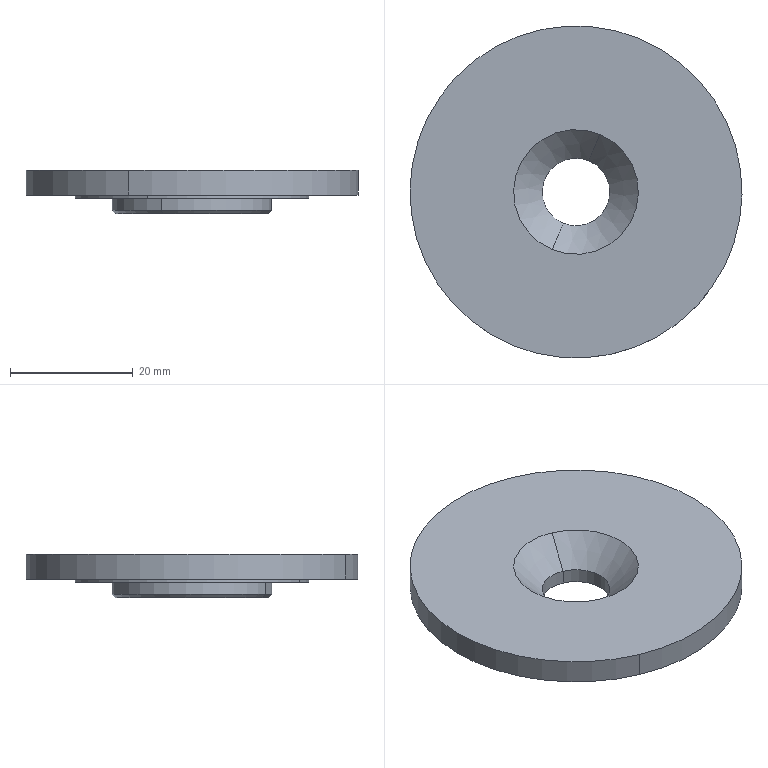Component | SolidWorks | 12AFlatGrooveSmallWheel-MillingAxis-1_12ASmallStraighteningWheelCover-1 | 1 solid | 16 faces | box 54 x 54 x 7 mm | volume 9901 mm3 | cylinder 8 | cone 4 | plane 4 | commonest cylinder face diameters 11 x2 54 x2 38 x2 26 x2 | material 45
build123d program:
from build123d import *

# Parameters (mm, degrees)
HOLE_SIZE_ACCORDING_TO_HEXAGON_SOCKET_D           = 11
HOLE_SIZE_ACCORDING_TO_HEXAGON_SOCKET_DEPTH       = 32.75
HOLE_SIZE_ACCORDING_TO_HEXAGON_SOCKET_CSINK_D     = 20.3
HOLE_SIZE_ACCORDING_TO_HEXAGON_SOCKET_CSINK_ANGLE = 90
HOLE_SIZE_ACCORDING_TO_HEXAGON_SOCKET_TIP         = 3.305
CHAMFER1_SIZE                                     = 0.5


with BuildPart() as part:
    # Sketch1 → Revolve1 (revolve)
    with BuildSketch(Plane.XY, mode=Mode.PRIVATE) as revolve1_sk:
        Polygon((0, 0), (0, 13), (2.5, 13), (2.5, 19), (3, 19), (3, 27), (7, 27), (7, 0), align=None)
    revolve(revolve1_sk.sketch.rotate(Axis((0, 0, 0), (1, 0, 0)), 90), axis=Axis((0, 0, 0), (1, 0, 0)))

    # Hole Size _ according to_ Hexagon Socket
    with Locations(Plane(origin=(7, 0, 0), x_dir=(0, 0, -1), z_dir=(1, 0, 0))):
        with Locations((0, 0)):
            CounterSinkHole(HOLE_SIZE_ACCORDING_TO_HEXAGON_SOCKET_D / 2, HOLE_SIZE_ACCORDING_TO_HEXAGON_SOCKET_CSINK_D / 2, depth=HOLE_SIZE_ACCORDING_TO_HEXAGON_SOCKET_DEPTH, counter_sink_angle=HOLE_SIZE_ACCORDING_TO_HEXAGON_SOCKET_CSINK_ANGLE)
            with Locations((0, 0, -(HOLE_SIZE_ACCORDING_TO_HEXAGON_SOCKET_DEPTH + HOLE_SIZE_ACCORDING_TO_HEXAGON_SOCKET_TIP / 2))):  # 118° drill point
                Cone(0, HOLE_SIZE_ACCORDING_TO_HEXAGON_SOCKET_D / 2, HOLE_SIZE_ACCORDING_TO_HEXAGON_SOCKET_TIP, mode=Mode.SUBTRACT)

    # Chamfer1
    chamfer1_edges = [part.edges().sort_by_distance(p)[0] for p in [
        (0, 0, -13),
    ]]
    chamfer(chamfer1_edges, length=CHAMFER1_SIZE)


solid = part.part

# Placed as in the assembly
solid = solid.moved(Location((-170.402, 66.538, 49.25), (0, -90, 0)))
STEP:
#1=CARTESIAN_POINT('',(-6.897,2.165,1.939));
#2=VERTEX_POINT('',#1);
#3=CARTESIAN_POINT('',(-6.521,3.074,1.939));
#4=VERTEX_POINT('',#3);
#5=CARTESIAN_POINT('',(-6.709,2.62,1.939));
#6=DIRECTION('',(0.,0.,-1.));
#7=DIRECTION('',(0.3818,0.9242,0.));
#8=AXIS2_PLACEMENT_3D('',#5,#6,#7);
#9=CIRCLE('',#8,0.4921);
#10=EDGE_CURVE('',#2,#4,#9,.T.);
#11=ORIENTED_EDGE('',*,*,#10,.F.);
#12=CARTESIAN_POINT('',(-6.904,2.147,1.959));
#13=VERTEX_POINT('',#12);
#14=CARTESIAN_POINT('',(-6.897,2.165,1.939));
#15=DIRECTION('',(-0.27,-0.6535,0.7071));
#16=VECTOR('',#15,39.37);
#17=LINE('',#14,#16);
#18=EDGE_CURVE('',#2,#13,#17,.T.);
#19=ORIENTED_EDGE('',*,*,#18,.T.);
#20=CARTESIAN_POINT('',(-6.513,3.093,1.959));
#21=VERTEX_POINT('',#20);
#22=CARTESIAN_POINT('',(-6.709,2.62,1.959));
#23=DIRECTION('',(0.,0.,1.));
#24=DIRECTION('',(0.3818,0.9242,0.));
#25=AXIS2_PLACEMENT_3D('',#22,#23,#24);
#26=CIRCLE('',#25,0.5118);
#27=EDGE_CURVE('',#21,#13,#26,.T.);
#28=ORIENTED_EDGE('',*,*,#27,.F.);
#29=CARTESIAN_POINT('',(-6.521,3.074,1.939));
#30=DIRECTION('',(0.27,0.6535,0.7071));
#31=VECTOR('',#30,39.37);
#32=LINE('',#29,#31);
#33=EDGE_CURVE('',#4,#21,#32,.T.);
#34=ORIENTED_EDGE('',*,*,#33,.F.);
#35=EDGE_LOOP('',(#11,#19,#28,#34));
#36=FACE_OUTER_BOUND('',#35,.T.);
#37=CARTESIAN_POINT('',(-6.709,2.62,1.939));
#38=DIRECTION('',(0.,0.,1.));
#39=DIRECTION('',(0.3818,0.9242,0.));
#40=AXIS2_PLACEMENT_3D('',#37,#38,#39);
#41=CONICAL_SURFACE('',#40,0.4921,0.7854);
#42=ADVANCED_FACE('',(#36),#41,.T.);
#43=CARTESIAN_POINT('',(-6.791,2.419,2.031));
#44=VERTEX_POINT('',#43);
#45=CARTESIAN_POINT('',(-6.626,2.82,2.031));
#46=VERTEX_POINT('',#45);
#47=CARTESIAN_POINT('',(-6.709,2.62,2.031));
#48=DIRECTION('',(0.,0.,1.));
#49=DIRECTION('',(0.3818,0.9242,0.));
#50=AXIS2_PLACEMENT_3D('',#47,#48,#49);
#51=CIRCLE('',#50,0.2165);
#52=EDGE_CURVE('',#44,#46,#51,.T.);
#53=ORIENTED_EDGE('',*,*,#52,.F.);
#54=CARTESIAN_POINT('',(-6.861,2.25,2.215));
#55=VERTEX_POINT('',#54);
#56=CARTESIAN_POINT('',(-6.861,2.25,2.215));
#57=DIRECTION('',(-0.27,-0.6535,0.7071));
#58=VECTOR('',#57,39.37);
#59=LINE('',#56,#58);
#60=EDGE_CURVE('',#44,#55,#59,.T.);
#61=ORIENTED_EDGE('',*,*,#60,.T.);
#62=CARTESIAN_POINT('',(-6.556,2.989,2.215));
#63=VERTEX_POINT('',#62);
#64=CARTESIAN_POINT('',(-6.709,2.62,2.215));
#65=DIRECTION('',(0.,0.,1.));
#66=DIRECTION('',(0.3818,0.9242,0.));
#67=AXIS2_PLACEMENT_3D('',#64,#65,#66);
#68=CIRCLE('',#67,0.3996);
#69=EDGE_CURVE('',#55,#63,#68,.T.);
#70=ORIENTED_EDGE('',*,*,#69,.T.);
#71=CARTESIAN_POINT('',(-6.556,2.989,2.215));
#72=DIRECTION('',(0.27,0.6535,0.7071));
#73=VECTOR('',#72,39.37);
#74=LINE('',#71,#73);
#75=EDGE_CURVE('',#46,#63,#74,.T.);
#76=ORIENTED_EDGE('',*,*,#75,.F.);
#77=EDGE_LOOP('',(#53,#61,#70,#76));
#78=FACE_OUTER_BOUND('',#77,.T.);
#79=CARTESIAN_POINT('',(-6.709,2.62,2.215));
#80=DIRECTION('',(0.,0.,1.));
#81=DIRECTION('',(0.3818,0.9242,0.));
#82=AXIS2_PLACEMENT_3D('',#79,#80,#81);
#83=CONICAL_SURFACE('',#82,0.3996,0.7854);
#84=ADVANCED_FACE('',(#78),#83,.F.);
#85=CARTESIAN_POINT('',(-6.791,2.419,1.939));
#86=VERTEX_POINT('',#85);
#87=CARTESIAN_POINT('',(-6.626,2.82,1.939));
#88=VERTEX_POINT('',#87);
#89=CARTESIAN_POINT('',(-6.709,2.62,1.939));
#90=DIRECTION('',(0.,0.,1.));
#91=DIRECTION('',(0.3818,0.9242,0.));
#92=AXIS2_PLACEMENT_3D('',#89,#90,#91);
#93=CIRCLE('',#92,0.2165);
#94=EDGE_CURVE('',#86,#88,#93,.T.);
#95=ORIENTED_EDGE('',*,*,#94,.F.);
#96=CARTESIAN_POINT('',(-6.791,2.419,2.215));
#97=DIRECTION('',(0.,0.,1.));
#98=VECTOR('',#97,39.37);
#99=LINE('',#96,#98);
#100=EDGE_CURVE('',#86,#44,#99,.T.);
#101=ORIENTED_EDGE('',*,*,#100,.T.);
#102=ORIENTED_EDGE('',*,*,#52,.T.);
#103=CARTESIAN_POINT('',(-6.626,2.82,2.215));
#104=DIRECTION('',(0.,0.,1.));
#105=VECTOR('',#104,39.37);
#106=LINE('',#103,#105);
#107=EDGE_CURVE('',#88,#46,#106,.T.);
#108=ORIENTED_EDGE('',*,*,#107,.F.);
#109=EDGE_LOOP('',(#95,#101,#102,#108));
#110=FACE_OUTER_BOUND('',#109,.T.);
#111=CARTESIAN_POINT('',(-6.709,2.62,2.215));
#112=DIRECTION('',(0.,0.,1.));
#113=DIRECTION('',(0.3818,0.9242,0.));
#114=AXIS2_PLACEMENT_3D('',#111,#112,#113);
#115=CYLINDRICAL_SURFACE('',#114,0.2165);
#116=ADVANCED_FACE('',(#110),#115,.F.);
#117=CARTESIAN_POINT('',(-7.115,1.637,2.215));
#118=VERTEX_POINT('',#117);
#119=CARTESIAN_POINT('',(-6.303,3.602,2.215));
#120=VERTEX_POINT('',#119);
#121=CARTESIAN_POINT('',(-6.709,2.62,2.215));
#122=DIRECTION('',(0.,0.,-1.));
#123=DIRECTION('',(-0.3818,-0.9242,0.));
#124=AXIS2_PLACEMENT_3D('',#121,#122,#123);
#125=CIRCLE('',#124,1.063);
#126=EDGE_CURVE('',#118,#120,#125,.T.);
#127=ORIENTED_EDGE('',*,*,#126,.T.);
#128=CARTESIAN_POINT('',(-6.303,3.602,2.057));
#129=VERTEX_POINT('',#128);
#130=CARTESIAN_POINT('',(-6.303,3.602,1.939));
#131=DIRECTION('',(0.,0.,-1.));
#132=VECTOR('',#131,39.37);
#133=LINE('',#130,#132);
#134=EDGE_CURVE('',#120,#129,#133,.T.);
#135=ORIENTED_EDGE('',*,*,#134,.T.);
#136=CARTESIAN_POINT('',(-7.115,1.637,2.057));
#137=VERTEX_POINT('',#136);
#138=CARTESIAN_POINT('',(-6.709,2.62,2.057));
#139=DIRECTION('',(0.,0.,-1.));
#140=DIRECTION('',(-0.3818,-0.9242,0.));
#141=AXIS2_PLACEMENT_3D('',#138,#139,#140);
#142=CIRCLE('',#141,1.063);
#143=EDGE_CURVE('',#137,#129,#142,.T.);
#144=ORIENTED_EDGE('',*,*,#143,.F.);
#145=CARTESIAN_POINT('',(-7.115,1.637,1.939));
#146=DIRECTION('',(0.,0.,-1.));
#147=VECTOR('',#146,39.37);
#148=LINE('',#145,#147);
#149=EDGE_CURVE('',#118,#137,#148,.T.);
#150=ORIENTED_EDGE('',*,*,#149,.F.);
#151=EDGE_LOOP('',(#127,#135,#144,#150));
#152=FACE_OUTER_BOUND('',#151,.T.);
#153=CARTESIAN_POINT('',(-6.709,2.62,1.939));
#154=DIRECTION('',(0.,0.,-1.));
#155=DIRECTION('',(-0.3818,-0.9242,0.));
#156=AXIS2_PLACEMENT_3D('',#153,#154,#155);
#157=CYLINDRICAL_SURFACE('',#156,1.063);
#158=ADVANCED_FACE('',(#152),#157,.T.);
#159=CARTESIAN_POINT('',(-6.994,1.928,2.057));
#160=VERTEX_POINT('',#159);
#161=CARTESIAN_POINT('',(-6.423,3.311,2.057));
#162=VERTEX_POINT('',#161);
#163=CARTESIAN_POINT('',(-6.709,2.62,2.057));
#164=DIRECTION('',(0.,0.,-1.));
#165=DIRECTION('',(-0.3818,-0.9242,0.));
#166=AXIS2_PLACEMENT_3D('',#163,#164,#165);
#167=CIRCLE('',#166,0.748);
#168=EDGE_CURVE('',#160,#162,#167,.T.);
#169=ORIENTED_EDGE('',*,*,#168,.T.);
#170=CARTESIAN_POINT('',(-6.423,3.311,2.037));
#171=VERTEX_POINT('',#170);
#172=CARTESIAN_POINT('',(-6.423,3.311,1.939));
#173=DIRECTION('',(0.,0.,-1.));
#174=VECTOR('',#173,39.37);
#175=LINE('',#172,#174);
#176=EDGE_CURVE('',#162,#171,#175,.T.);
#177=ORIENTED_EDGE('',*,*,#176,.T.);
#178=CARTESIAN_POINT('',(-6.994,1.928,2.037));
#179=VERTEX_POINT('',#178);
#180=CARTESIAN_POINT('',(-6.709,2.62,2.037));
#181=DIRECTION('',(0.,0.,-1.));
#182=DIRECTION('',(-0.3818,-0.9242,0.));
#183=AXIS2_PLACEMENT_3D('',#180,#181,#182);
#184=CIRCLE('',#183,0.748);
#185=EDGE_CURVE('',#179,#171,#184,.T.);
#186=ORIENTED_EDGE('',*,*,#185,.F.);
#187=CARTESIAN_POINT('',(-6.994,1.928,1.939));
#188=DIRECTION('',(0.,0.,-1.));
#189=VECTOR('',#188,39.37);
#190=LINE('',#187,#189);
#191=EDGE_CURVE('',#160,#179,#190,.T.);
#192=ORIENTED_EDGE('',*,*,#191,.F.);
#193=EDGE_LOOP('',(#169,#177,#186,#192));
#194=FACE_OUTER_BOUND('',#193,.T.);
#195=CARTESIAN_POINT('',(-6.709,2.62,1.939));
#196=DIRECTION('',(0.,0.,-1.));
#197=DIRECTION('',(-0.3818,-0.9242,0.));
#198=AXIS2_PLACEMENT_3D('',#195,#196,#197);
#199=CYLINDRICAL_SURFACE('',#198,0.748);
#200=ADVANCED_FACE('',(#194),#199,.T.);
#201=CARTESIAN_POINT('',(-6.904,2.147,2.037));
#202=VERTEX_POINT('',#201);
#203=CARTESIAN_POINT('',(-6.513,3.093,2.037));
#204=VERTEX_POINT('',#203);
#205=CARTESIAN_POINT('',(-6.709,2.62,2.037));
#206=DIRECTION('',(0.,0.,-1.));
#207=DIRECTION('',(-0.3818,-0.9242,0.));
#208=AXIS2_PLACEMENT_3D('',#205,#206,#207);
#209=CIRCLE('',#208,0.5118);
#210=EDGE_CURVE('',#202,#204,#209,.T.);
#211=ORIENTED_EDGE('',*,*,#210,.T.);
#212=CARTESIAN_POINT('',(-6.513,3.093,1.939));
#213=DIRECTION('',(0.,0.,-1.));
#214=VECTOR('',#213,39.37);
#215=LINE('',#212,#214);
#216=EDGE_CURVE('',#204,#21,#215,.T.);
#217=ORIENTED_EDGE('',*,*,#216,.T.);
#218=ORIENTED_EDGE('',*,*,#27,.T.);
#219=CARTESIAN_POINT('',(-6.904,2.147,1.939));
#220=DIRECTION('',(0.,0.,-1.));
#221=VECTOR('',#220,39.37);
#222=LINE('',#219,#221);
#223=EDGE_CURVE('',#202,#13,#222,.T.);
#224=ORIENTED_EDGE('',*,*,#223,.F.);
#225=EDGE_LOOP('',(#211,#217,#218,#224));
#226=FACE_OUTER_BOUND('',#225,.T.);
#227=CARTESIAN_POINT('',(-6.709,2.62,1.939));
#228=DIRECTION('',(0.,0.,-1.));
#229=DIRECTION('',(-0.3818,-0.9242,0.));
#230=AXIS2_PLACEMENT_3D('',#227,#228,#229);
#231=CYLINDRICAL_SURFACE('',#230,0.5118);
#232=ADVANCED_FACE('',(#226),#231,.T.);
#233=CARTESIAN_POINT('',(-6.709,2.62,1.939));
#234=DIRECTION('',(0.,0.,-1.));
#235=DIRECTION('',(0.3818,0.9242,0.));
#236=AXIS2_PLACEMENT_3D('',#233,#234,#235);
#237=CIRCLE('',#236,0.4921);
#238=EDGE_CURVE('',#4,#2,#237,.T.);
#239=ORIENTED_EDGE('',*,*,#238,.T.);
#240=ORIENTED_EDGE('',*,*,#10,.T.);
#241=EDGE_LOOP('',(#239,#240));
#242=FACE_OUTER_BOUND('',#241,.T.);
#243=CARTESIAN_POINT('',(-6.709,2.62,1.939));
#244=DIRECTION('',(0.,0.,1.));
#245=DIRECTION('',(0.3818,0.9242,0.));
#246=AXIS2_PLACEMENT_3D('',#243,#244,#245);
#247=CIRCLE('',#246,0.2165);
#248=EDGE_CURVE('',#88,#86,#247,.T.);
#249=ORIENTED_EDGE('',*,*,#248,.T.);
#250=ORIENTED_EDGE('',*,*,#94,.T.);
#251=EDGE_LOOP('',(#249,#250));
#252=FACE_BOUND('',#251,.T.);
#253=CARTESIAN_POINT('',(-6.709,2.62,1.939));
#254=DIRECTION('',(0.,0.,1.));
#255=DIRECTION('',(0.3818,0.9242,0.));
#256=AXIS2_PLACEMENT_3D('',#253,#254,#255);
#257=PLANE('',#256);
#258=ADVANCED_FACE('',(#242,#252),#257,.F.);
#259=ORIENTED_EDGE('',*,*,#216,.F.);
#260=CARTESIAN_POINT('',(-6.709,2.62,2.037));
#261=DIRECTION('',(0.,0.,-1.));
#262=DIRECTION('',(-0.3818,-0.9242,0.));
#263=AXIS2_PLACEMENT_3D('',#260,#261,#262);
#264=CIRCLE('',#263,0.5118);
#265=EDGE_CURVE('',#204,#202,#264,.T.);
#266=ORIENTED_EDGE('',*,*,#265,.T.);
#267=ORIENTED_EDGE('',*,*,#223,.T.);
#268=CARTESIAN_POINT('',(-6.709,2.62,1.959));
#269=DIRECTION('',(0.,0.,1.));
#270=DIRECTION('',(0.3818,0.9242,0.));
#271=AXIS2_PLACEMENT_3D('',#268,#269,#270);
#272=CIRCLE('',#271,0.5118);
#273=EDGE_CURVE('',#13,#21,#272,.T.);
#274=ORIENTED_EDGE('',*,*,#273,.T.);
#275=EDGE_LOOP('',(#259,#266,#267,#274));
#276=FACE_OUTER_BOUND('',#275,.T.);
#277=CARTESIAN_POINT('',(-6.709,2.62,1.939));
#278=DIRECTION('',(0.,0.,-1.));
#279=DIRECTION('',(-0.3818,-0.9242,0.));
#280=AXIS2_PLACEMENT_3D('',#277,#278,#279);
#281=CYLINDRICAL_SURFACE('',#280,0.5118);
#282=ADVANCED_FACE('',(#276),#281,.T.);
#283=ORIENTED_EDGE('',*,*,#210,.F.);
#284=ORIENTED_EDGE('',*,*,#265,.F.);
#285=EDGE_LOOP('',(#283,#284));
#286=FACE_BOUND('',#285,.T.);
#287=ORIENTED_EDGE('',*,*,#185,.T.);
#288=CARTESIAN_POINT('',(-6.709,2.62,2.037));
#289=DIRECTION('',(0.,0.,-1.));
#290=DIRECTION('',(-0.3818,-0.9242,0.));
#291=AXIS2_PLACEMENT_3D('',#288,#289,#290);
#292=CIRCLE('',#291,0.748);
#293=EDGE_CURVE('',#171,#179,#292,.T.);
#294=ORIENTED_EDGE('',*,*,#293,.T.);
#295=EDGE_LOOP('',(#287,#294));
#296=FACE_OUTER_BOUND('',#295,.T.);
#297=CARTESIAN_POINT('',(-7.182,2.815,2.037));
#298=DIRECTION('',(0.,0.,1.));
#299=DIRECTION('',(0.3818,0.9242,0.));
#300=AXIS2_PLACEMENT_3D('',#297,#298,#299);
#301=PLANE('',#300);
#302=ADVANCED_FACE('',(#286,#296),#301,.F.);
#303=ORIENTED_EDGE('',*,*,#176,.F.);
#304=CARTESIAN_POINT('',(-6.709,2.62,2.057));
#305=DIRECTION('',(0.,0.,-1.));
#306=DIRECTION('',(-0.3818,-0.9242,0.));
#307=AXIS2_PLACEMENT_3D('',#304,#305,#306);
#308=CIRCLE('',#307,0.748);
#309=EDGE_CURVE('',#162,#160,#308,.T.);
#310=ORIENTED_EDGE('',*,*,#309,.T.);
#311=ORIENTED_EDGE('',*,*,#191,.T.);
#312=ORIENTED_EDGE('',*,*,#293,.F.);
#313=EDGE_LOOP('',(#303,#310,#311,#312));
#314=FACE_OUTER_BOUND('',#313,.T.);
#315=CARTESIAN_POINT('',(-6.709,2.62,1.939));
#316=DIRECTION('',(0.,0.,-1.));
#317=DIRECTION('',(-0.3818,-0.9242,0.));
#318=AXIS2_PLACEMENT_3D('',#315,#316,#317);
#319=CYLINDRICAL_SURFACE('',#318,0.748);
#320=ADVANCED_FACE('',(#314),#319,.T.);
#321=ORIENTED_EDGE('',*,*,#168,.F.);
#322=ORIENTED_EDGE('',*,*,#309,.F.);
#323=EDGE_LOOP('',(#321,#322));
#324=FACE_BOUND('',#323,.T.);
#325=ORIENTED_EDGE('',*,*,#143,.T.);
#326=CARTESIAN_POINT('',(-6.709,2.62,2.057));
#327=DIRECTION('',(0.,0.,-1.));
#328=DIRECTION('',(-0.3818,-0.9242,0.));
#329=AXIS2_PLACEMENT_3D('',#326,#327,#328);
#330=CIRCLE('',#329,1.063);
#331=EDGE_CURVE('',#129,#137,#330,.T.);
#332=ORIENTED_EDGE('',*,*,#331,.T.);
#333=EDGE_LOOP('',(#325,#332));
#334=FACE_OUTER_BOUND('',#333,.T.);
#335=CARTESIAN_POINT('',(-7.4,2.905,2.057));
#336=DIRECTION('',(0.,0.,1.));
#337=DIRECTION('',(0.3818,0.9242,0.));
#338=AXIS2_PLACEMENT_3D('',#335,#336,#337);
#339=PLANE('',#338);
#340=ADVANCED_FACE('',(#324,#334),#339,.F.);
#341=ORIENTED_EDGE('',*,*,#134,.F.);
#342=CARTESIAN_POINT('',(-6.709,2.62,2.215));
#343=DIRECTION('',(0.,0.,-1.));
#344=DIRECTION('',(-0.3818,-0.9242,0.));
#345=AXIS2_PLACEMENT_3D('',#342,#343,#344);
#346=CIRCLE('',#345,1.063);
#347=EDGE_CURVE('',#120,#118,#346,.T.);
#348=ORIENTED_EDGE('',*,*,#347,.T.);
#349=ORIENTED_EDGE('',*,*,#149,.T.);
#350=ORIENTED_EDGE('',*,*,#331,.F.);
#351=EDGE_LOOP('',(#341,#348,#349,#350));
#352=FACE_OUTER_BOUND('',#351,.T.);
#353=CARTESIAN_POINT('',(-6.709,2.62,1.939));
#354=DIRECTION('',(0.,0.,-1.));
#355=DIRECTION('',(-0.3818,-0.9242,0.));
#356=AXIS2_PLACEMENT_3D('',#353,#354,#355);
#357=CYLINDRICAL_SURFACE('',#356,1.063);
#358=ADVANCED_FACE('',(#352),#357,.T.);
#359=CARTESIAN_POINT('',(-6.709,2.62,2.215));
#360=DIRECTION('',(0.,0.,1.));
#361=DIRECTION('',(0.3818,0.9242,0.));
#362=AXIS2_PLACEMENT_3D('',#359,#360,#361);
#363=CIRCLE('',#362,0.3996);
#364=EDGE_CURVE('',#63,#55,#363,.T.);
#365=ORIENTED_EDGE('',*,*,#364,.F.);
#366=ORIENTED_EDGE('',*,*,#69,.F.);
#367=EDGE_LOOP('',(#365,#366));
#368=FACE_BOUND('',#367,.T.);
#369=ORIENTED_EDGE('',*,*,#126,.F.);
#370=ORIENTED_EDGE('',*,*,#347,.F.);
#371=EDGE_LOOP('',(#369,#370));
#372=FACE_OUTER_BOUND('',#371,.T.);
#373=CARTESIAN_POINT('',(-7.691,3.026,2.215));
#374=DIRECTION('',(0.,0.,-1.));
#375=DIRECTION('',(-0.3818,-0.9242,0.));
#376=AXIS2_PLACEMENT_3D('',#373,#374,#375);
#377=PLANE('',#376);
#378=ADVANCED_FACE('',(#368,#372),#377,.F.);
#379=ORIENTED_EDGE('',*,*,#100,.F.);
#380=ORIENTED_EDGE('',*,*,#248,.F.);
#381=ORIENTED_EDGE('',*,*,#107,.T.);
#382=CARTESIAN_POINT('',(-6.709,2.62,2.031));
#383=DIRECTION('',(0.,0.,1.));
#384=DIRECTION('',(0.3818,0.9242,0.));
#385=AXIS2_PLACEMENT_3D('',#382,#383,#384);
#386=CIRCLE('',#385,0.2165);
#387=EDGE_CURVE('',#46,#44,#386,.T.);
#388=ORIENTED_EDGE('',*,*,#387,.T.);
#389=EDGE_LOOP('',(#379,#380,#381,#388));
#390=FACE_OUTER_BOUND('',#389,.T.);
#391=CARTESIAN_POINT('',(-6.709,2.62,2.215));
#392=DIRECTION('',(0.,0.,1.));
#393=DIRECTION('',(0.3818,0.9242,0.));
#394=AXIS2_PLACEMENT_3D('',#391,#392,#393);
#395=CYLINDRICAL_SURFACE('',#394,0.2165);
#396=ADVANCED_FACE('',(#390),#395,.F.);
#397=ORIENTED_EDGE('',*,*,#60,.F.);
#398=ORIENTED_EDGE('',*,*,#387,.F.);
#399=ORIENTED_EDGE('',*,*,#75,.T.);
#400=ORIENTED_EDGE('',*,*,#364,.T.);
#401=EDGE_LOOP('',(#397,#398,#399,#400));
#402=FACE_OUTER_BOUND('',#401,.T.);
#403=CARTESIAN_POINT('',(-6.709,2.62,2.215));
#404=DIRECTION('',(0.,0.,1.));
#405=DIRECTION('',(0.3818,0.9242,0.));
#406=AXIS2_PLACEMENT_3D('',#403,#404,#405);
#407=CONICAL_SURFACE('',#406,0.3996,0.7854);
#408=ADVANCED_FACE('',(#402),#407,.F.);
#409=ORIENTED_EDGE('',*,*,#18,.F.);
#410=ORIENTED_EDGE('',*,*,#238,.F.);
#411=ORIENTED_EDGE('',*,*,#33,.T.);
#412=ORIENTED_EDGE('',*,*,#273,.F.);
#413=EDGE_LOOP('',(#409,#410,#411,#412));
#414=FACE_OUTER_BOUND('',#413,.T.);
#415=CARTESIAN_POINT('',(-6.709,2.62,1.939));
#416=DIRECTION('',(0.,0.,1.));
#417=DIRECTION('',(0.3818,0.9242,0.));
#418=AXIS2_PLACEMENT_3D('',#415,#416,#417);
#419=CONICAL_SURFACE('',#418,0.4921,0.7854);
#420=ADVANCED_FACE('',(#414),#419,.T.);
#421=CLOSED_SHELL('',(#42,#84,#116,#158,#200,#232,#258,#282,#302,#320,#340,#358,#378,#396,#408,#420));
#422=MANIFOLD_SOLID_BREP('',#421);
#423=CARTESIAN_POINT('',(0.,0.,0.));
#424=DIRECTION('',(0.,0.,1.));
#425=DIRECTION('',(1.,0.,0.));
#426=AXIS2_PLACEMENT_3D('',#423,#424,#425);
#427=(LENGTH_UNIT()NAMED_UNIT(*)SI_UNIT($,.METRE.));
#428=LENGTH_MEASURE_WITH_UNIT(LENGTH_MEASURE(0.0254),#427);
#429=DIMENSIONAL_EXPONENTS(1.,0.,0.,0.,0.,0.,0.);
#430=(CONVERSION_BASED_UNIT('',#428)LENGTH_UNIT()NAMED_UNIT(#429));
#431=UNCERTAINTY_MEASURE_WITH_UNIT(LENGTH_MEASURE(0.00001),#430,'','');
#432=(NAMED_UNIT(*)PLANE_ANGLE_UNIT()SI_UNIT($,.RADIAN.));
#433=(NAMED_UNIT(*)SI_UNIT($,.STERADIAN.)SOLID_ANGLE_UNIT());
#434=(GEOMETRIC_REPRESENTATION_CONTEXT(3)GLOBAL_UNCERTAINTY_ASSIGNED_CONTEXT((#431))GLOBAL_UNIT_ASSIGNED_CONTEXT((#430,#432,#433))REPRESENTATION_CONTEXT('',''));
#435=ADVANCED_BREP_SHAPE_REPRESENTATION('',(#422,#426),#434);
#436=COLOUR_RGB('',0.7922,0.8196,0.9333);
#437=FILL_AREA_STYLE_COLOUR('',#436);
#438=FILL_AREA_STYLE('',(#437));
#439=SURFACE_STYLE_FILL_AREA(#438);
#440=SURFACE_SIDE_STYLE('',(#439));
#441=SURFACE_STYLE_USAGE(.BOTH.,#440);
#442=PRESENTATION_STYLE_ASSIGNMENT((#441));
#443=STYLED_ITEM('',(#442),#422);
#444=(LENGTH_UNIT()NAMED_UNIT(*)SI_UNIT($,.METRE.));
#445=LENGTH_MEASURE_WITH_UNIT(LENGTH_MEASURE(0.0254),#444);
#446=DIMENSIONAL_EXPONENTS(1.,0.,0.,0.,0.,0.,0.);
#447=(CONVERSION_BASED_UNIT('',#445)LENGTH_UNIT()NAMED_UNIT(#446));
#448=UNCERTAINTY_MEASURE_WITH_UNIT(LENGTH_MEASURE(0.00001),#447,'','');
#449=(NAMED_UNIT(*)PLANE_ANGLE_UNIT()SI_UNIT($,.RADIAN.));
#450=(NAMED_UNIT(*)SI_UNIT($,.STERADIAN.)SOLID_ANGLE_UNIT());
#451=(GEOMETRIC_REPRESENTATION_CONTEXT(3)GLOBAL_UNCERTAINTY_ASSIGNED_CONTEXT((#448))GLOBAL_UNIT_ASSIGNED_CONTEXT((#447,#449,#450))REPRESENTATION_CONTEXT('',''));
#452=MECHANICAL_DESIGN_GEOMETRIC_PRESENTATION_REPRESENTATION('',(#443),#451);
#453=PRESENTATION_LAYER_ASSIGNMENT('','',(#443));